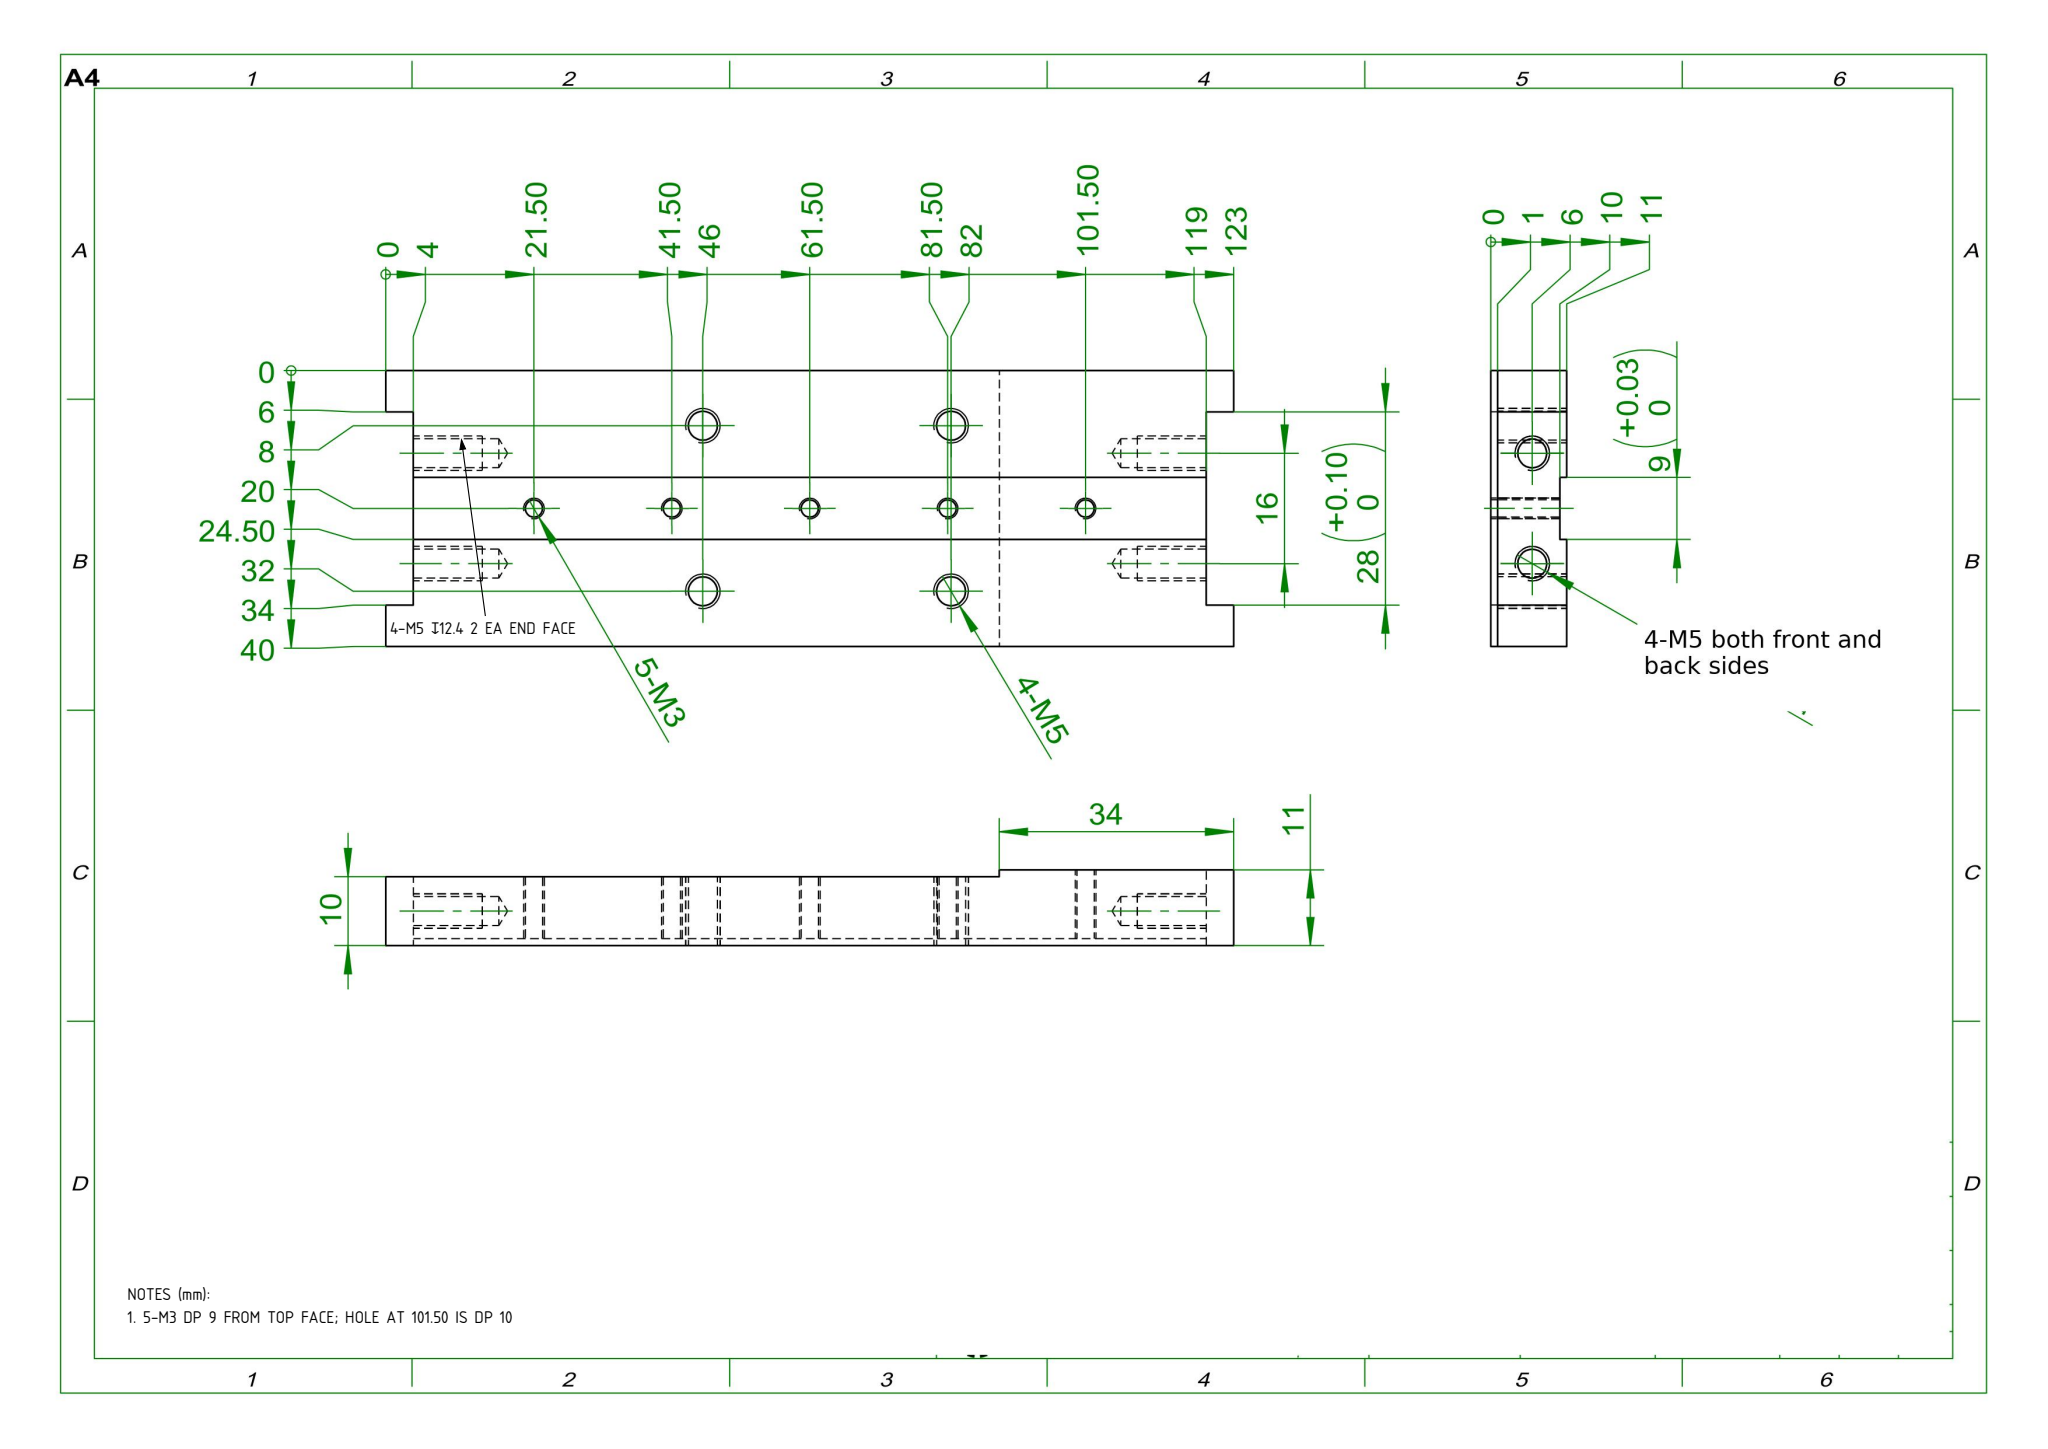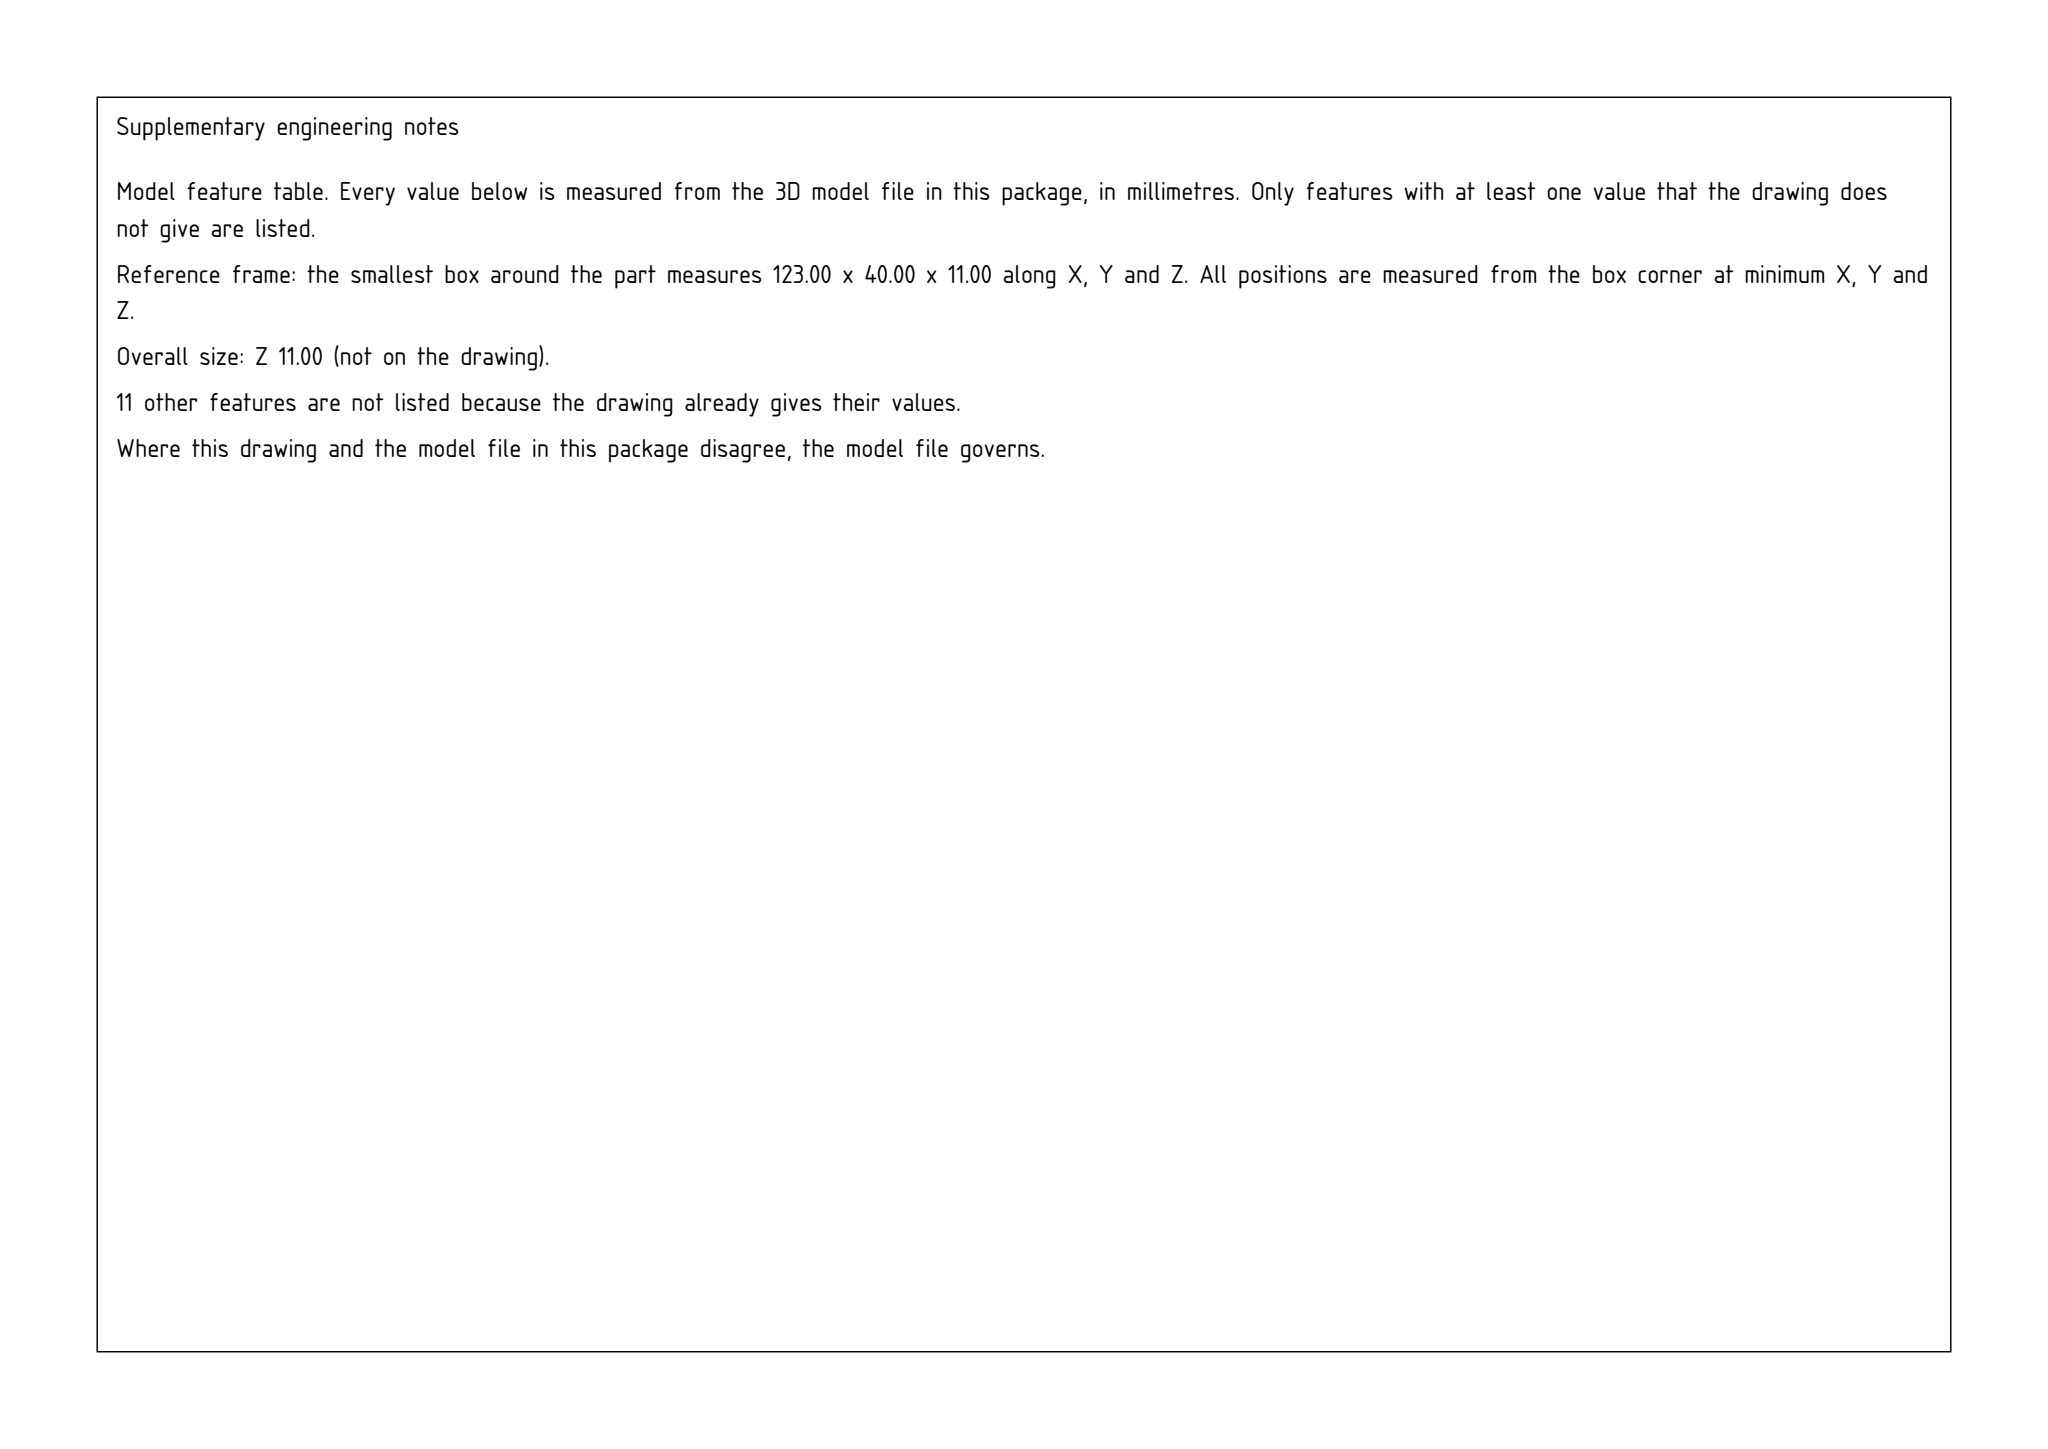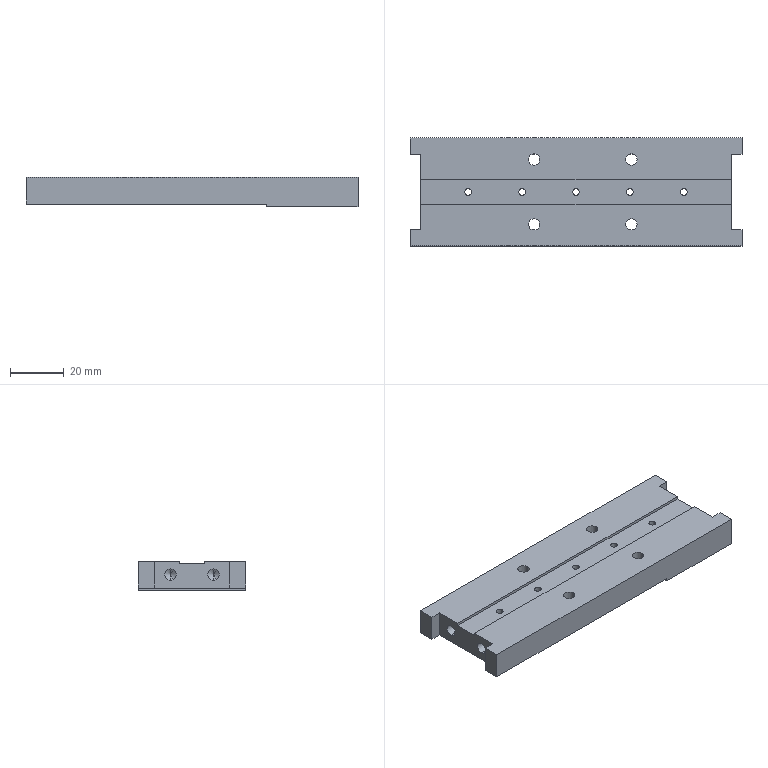Part | SolidWorks | mm | 1 solid | 54 faces | box 123 x 40 x 11 mm | volume 45683 mm3 | cylinder 26 | plane 20 | cone 8 | commonest cylinder face diameters 4.2 x16 2.5 x10
Drawing notes:
5-M3 DP 9 FROM TOP FACE; HOLE AT 101.50 IS DP 10 | from the solid: Ø2.5 z-axis cylinders at y=20, x=21.5/41.5/61.5/81.5 len 9.0; x=101.5 len 10.0 (M3 tap drill)
4-M5 DP 12.4, 2 EA END FACE (0 & 123), Y=12 & 28, Z=6 | from the solid: Ø4.2 x-axis cylinders at (y12,z6) and (y28,z6), length 12.4, from x=0 and x=123 faces
build123d program:
from build123d import *

# Parameters (mm, degrees)
SKETCH1_W             = 115
SKETCH1_H             = 40
BOSS_EXTRUDE1_DEPTH   = 10
SKETCH2_W             = 115
SKETCH2_H             = 9
CUT_EXTRUDE1_DEPTH    = 1
SKETCH3_W             = 30
SKETCH3_H             = 40
BOSS_EXTRUDE2_DEPTH   = 1
M5_TAPPED_HOLE1_D     = 4.2
M5_TAPPED_HOLE2_D     = 4.2
M5_TAPPED_HOLE2_DEPTH = 12.4
M5_TAPPED_HOLE2_TIP   = 1.262
M5_TAPPED_HOLE3_D     = 4.2
M5_TAPPED_HOLE3_DEPTH = 12.4
M5_TAPPED_HOLE3_TIP   = 1.262
M3_TAPPED_HOLE1_D     = 2.5
SKETCH14_W            = 10
SKETCH14_H            = 6
BOSS_EXTRUDE3_DEPTH   = 4
SKETCH15_W            = 11
SKETCH15_H            = 6
BOSS_EXTRUDE4_DEPTH   = 4


with BuildPart() as part:
    # Sketch1 → Boss-Extrude1 (new body)
    with BuildSketch(Plane.XY):
        Rectangle(SKETCH1_W, SKETCH1_H)
    extrude(amount=BOSS_EXTRUDE1_DEPTH)

    # Sketch2 → Cut-Extrude1 (cut)
    with BuildSketch(Plane.XY.offset(10)):
        Rectangle(SKETCH2_W, SKETCH2_H)
    extrude(amount=-CUT_EXTRUDE1_DEPTH, mode=Mode.SUBTRACT)

    # Sketch3 → Boss-Extrude2 (add)
    with BuildSketch(Plane(origin=(0, 0, 0), x_dir=(-1, 0, 0), z_dir=(0, 0, -1))):
        with Locations((-42.5, 0)):
            Rectangle(SKETCH3_W, SKETCH3_H)
    extrude(amount=BOSS_EXTRUDE2_DEPTH)

    # M5 Tapped Hole1 (through all)
    with Locations(Plane(origin=(0, 0, 0), x_dir=(-1, 0, 0), z_dir=(0, 0, -1))):
        with Locations((-20.5, 12), (15.5, 12), (15.5, -12), (-20.5, -12)):
            Hole(M5_TAPPED_HOLE1_D / 2)

    # M5 Tapped Hole2
    with Locations(Plane(origin=(57.5, 0, 0), x_dir=(0, 0, -1), z_dir=(1, 0, 0))):
        with Locations((-5, 8), (-5, -8)):
            Hole(M5_TAPPED_HOLE2_D / 2, depth=M5_TAPPED_HOLE2_DEPTH)
            with Locations((0, 0, -(M5_TAPPED_HOLE2_DEPTH + M5_TAPPED_HOLE2_TIP / 2))):  # 118° drill point
                Cone(0, M5_TAPPED_HOLE2_D / 2, M5_TAPPED_HOLE2_TIP, mode=Mode.SUBTRACT)

    # M5 Tapped Hole3
    with Locations(Plane.ZY.offset(57.5)):
        with Locations((5, 8), (5, -8)):
            Hole(M5_TAPPED_HOLE3_D / 2, depth=M5_TAPPED_HOLE3_DEPTH)
            with Locations((0, 0, -(M5_TAPPED_HOLE3_DEPTH + M5_TAPPED_HOLE3_TIP / 2))):  # 118° drill point
                Cone(0, M5_TAPPED_HOLE3_D / 2, M5_TAPPED_HOLE3_TIP, mode=Mode.SUBTRACT)

    # M3 Tapped Hole1 (through all)
    with Locations(Plane.XY.offset(9)):
        with Locations((-40, 0), (-20, 0), (0, 0), (20, 0), (40, 0)):
            Hole(M3_TAPPED_HOLE1_D / 2)

    # Sketch14 → Boss-Extrude3 (add)
    with BuildSketch(Plane.ZY.offset(57.5)):
        with Locations((5, 17)):
            Rectangle(SKETCH14_W, SKETCH14_H)
        with Locations((5, -17)):
            Rectangle(SKETCH14_W, SKETCH14_H)
    extrude(amount=BOSS_EXTRUDE3_DEPTH)

    # Sketch15 → Boss-Extrude4 (add)
    with BuildSketch(Plane(origin=(57.5, 0, 0), x_dir=(0, 0, -1), z_dir=(1, 0, 0))):
        with Locations((-4.5, 17)):
            Rectangle(SKETCH15_W, SKETCH15_H)
        with Locations((-4.5, -17)):
            Rectangle(SKETCH15_W, SKETCH15_H)
    extrude(amount=BOSS_EXTRUDE4_DEPTH)


solid = part.part